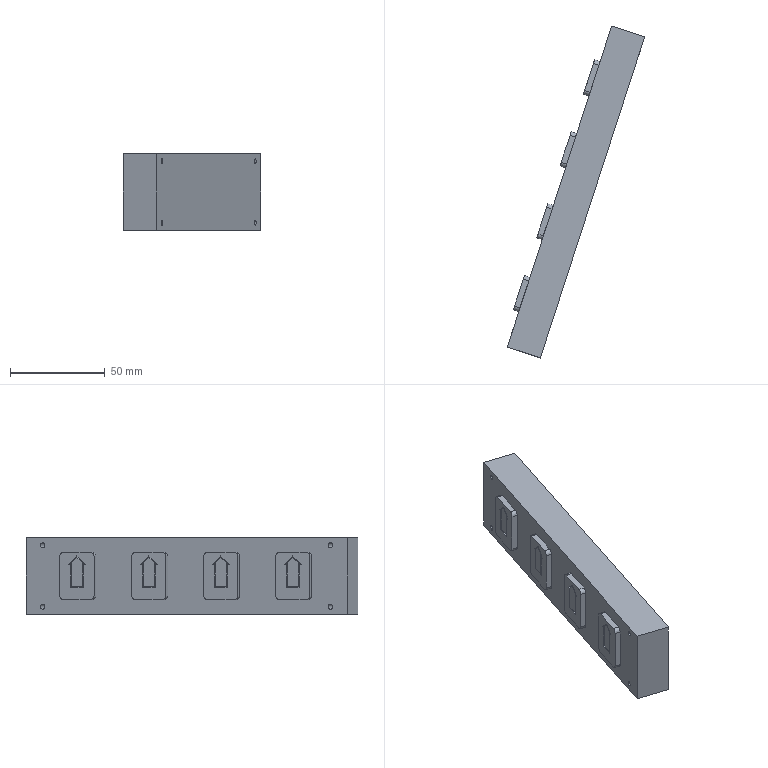Component | SolidWorks | DisplayPanel-1_NavigationKey-1 | 1 solid | 114 faces | box 72.75 x 175.48 x 40.5 mm | volume 138949 mm3 | plane 90 | cylinder 24 | commonest cylinder face diameters 4 x16 2.5 x8
build123d program:
from build123d import *

# Parameters (mm, degrees)
SKETCH1_W           = 40.5
SKETCH1_H           = 178.5
SKETCH1_R           = 1.25
BOSS_EXTRUDE1_DEPTH = 18.5
BOSS_EXTRUDE2_DEPTH = 3
CUT_EXTRUDE1_DEPTH  = 1
LPATTERN1_COUNT     = 4
LPATTERN1_PITCH     = 40


with BuildPart() as part:
    # Sketch1 → Boss-Extrude1 (new body)
    with BuildSketch(Plane.XY):
        with Locations((2340.361, 332.483)):
            Rectangle(SKETCH1_W, SKETCH1_H)
        with Locations((2324.111, 412.483)):
            Circle(SKETCH1_R, mode=Mode.SUBTRACT)
        with Locations((2356.611, 412.483)):
            Circle(SKETCH1_R, mode=Mode.SUBTRACT)
        with Locations((2356.611, 252.483)):
            Circle(SKETCH1_R, mode=Mode.SUBTRACT)
        with Locations((2324.111, 252.483)):
            Circle(SKETCH1_R, mode=Mode.SUBTRACT)
    extrude(amount=BOSS_EXTRUDE1_DEPTH)

    # Sketch2 → Boss-Extrude2 (add)
    with BuildSketch(Plane.XY.offset(18.5)):
        with BuildLine():
            Line((2350.861, 262.983), (2329.861, 262.983))
            ThreePointArc((2329.861, 262.983), (2328.447, 263.569), (2327.861, 264.983))
            Line((2327.861, 264.983), (2327.861, 279.983))
            ThreePointArc((2327.861, 279.983), (2328.447, 281.398), (2329.861, 281.983))
            Line((2329.861, 281.983), (2350.861, 281.983))
            ThreePointArc((2350.861, 281.983), (2352.275, 281.398), (2352.861, 279.983))
            Line((2352.861, 279.983), (2352.861, 264.983))
            ThreePointArc((2352.861, 264.983), (2352.275, 263.569), (2350.861, 262.983))
        make_face()
        with BuildLine():
            Line((2350.861, 302.983), (2329.861, 302.983))
            ThreePointArc((2329.861, 302.983), (2328.447, 303.569), (2327.861, 304.983))
            Line((2327.861, 304.983), (2327.861, 319.983))
            ThreePointArc((2327.861, 319.983), (2328.447, 321.398), (2329.861, 321.983))
            Line((2329.861, 321.983), (2350.861, 321.983))
            ThreePointArc((2350.861, 321.983), (2352.275, 321.398), (2352.861, 319.983))
            Line((2352.861, 319.983), (2352.861, 304.983))
            ThreePointArc((2352.861, 304.983), (2352.275, 303.569), (2350.861, 302.983))
        make_face()
        with BuildLine():
            Line((2350.861, 342.983), (2329.861, 342.983))
            ThreePointArc((2329.861, 342.983), (2328.447, 343.569), (2327.861, 344.983))
            Line((2327.861, 344.983), (2327.861, 359.983))
            ThreePointArc((2327.861, 359.983), (2328.447, 361.398), (2329.861, 361.983))
            Line((2329.861, 361.983), (2350.861, 361.983))
            ThreePointArc((2350.861, 361.983), (2352.275, 361.398), (2352.861, 359.983))
            Line((2352.861, 359.983), (2352.861, 344.983))
            ThreePointArc((2352.861, 344.983), (2352.275, 343.569), (2350.861, 342.983))
        make_face()
        with BuildLine():
            Line((2350.861, 382.983), (2329.861, 382.983))
            ThreePointArc((2329.861, 382.983), (2328.447, 383.569), (2327.861, 384.983))
            Line((2327.861, 384.983), (2327.861, 399.983))
            ThreePointArc((2327.861, 399.983), (2328.447, 401.398), (2329.861, 401.983))
            Line((2329.861, 401.983), (2350.861, 401.983))
            ThreePointArc((2350.861, 401.983), (2352.275, 401.398), (2352.861, 399.983))
            Line((2352.861, 399.983), (2352.861, 384.983))
            ThreePointArc((2352.861, 384.983), (2352.275, 383.569), (2350.861, 382.983))
        make_face()
    extrude(amount=BOSS_EXTRUDE2_DEPTH)

    # Sketch3 → Cut-Extrude1 (cut)
    with BuildSketch(Plane.XY.offset(21.5)):
        Polygon((2350.984, 392.483), (2346.34, 397.291), (2346.34, 395.971), (2334.382, 395.971), (2334.382, 388.995), (2346.34, 388.995), (2346.34, 387.675), align=None)
        Polygon((2350.289, 392.483), (2346.84, 396.054), (2346.84, 395.471), (2334.882, 395.471), (2334.882, 389.495), (2346.84, 389.495), (2346.84, 388.913), align=None, mode=Mode.SUBTRACT)
    cut_extrude1 = extrude(amount=-CUT_EXTRUDE1_DEPTH, mode=Mode.SUBTRACT)

    # LPattern1: Cut-Extrude1 ×4
    with Locations(*[(0, -i * LPATTERN1_PITCH, 0) for i in range(1, LPATTERN1_COUNT)]):
        add(cut_extrude1, mode=Mode.SUBTRACT)


solid = part.part

# Placed as in the assembly
solid = solid.moved(Location((51.937, -352.862, -2532.361), (-90, -72, -90)))